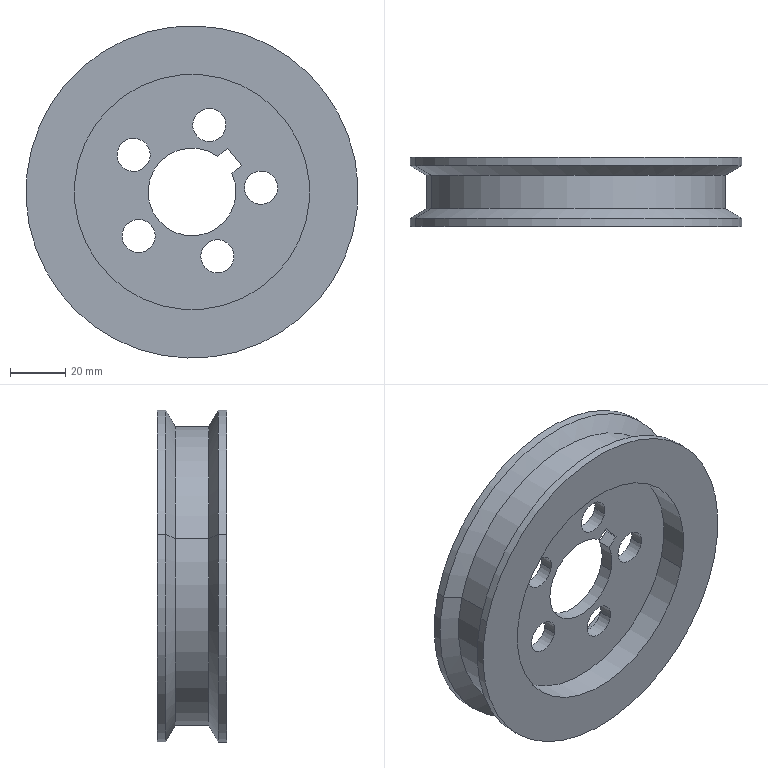Component | SolidWorks | LX-TSJ-04-1 | 1 solid | 34 faces | box 120 x 25 x 120 mm | volume 128781 mm3 | cylinder 23 | plane 7 | cone 4 | commonest cylinder face diameters 12 x10 120 x4 85 x4 31.75 x3 108 x2
STEP:
#1=CARTESIAN_POINT('',(-5.449,-19.146,-16.155));
#2=VERTEX_POINT('',#1);
#3=CARTESIAN_POINT('',(-4.238,-19.146,-16.467));
#4=VERTEX_POINT('',#3);
#5=CARTESIAN_POINT('',(-4.843,-19.146,-16.311));
#6=DIRECTION('',(0.,-1.,-0.));
#7=DIRECTION('',(0.9682,0.,-0.2502));
#8=AXIS2_PLACEMENT_3D('',#5,#6,#7);
#9=CIRCLE('',#8,0.625);
#10=EDGE_CURVE('',#2,#4,#9,.T.);
#11=ORIENTED_EDGE('',*,*,#10,.T.);
#12=CARTESIAN_POINT('',(-4.238,-18.949,-16.467));
#13=VERTEX_POINT('',#12);
#14=CARTESIAN_POINT('',(-4.238,-19.539,-16.467));
#15=DIRECTION('',(-0.,1.,0.));
#16=VECTOR('',#15,39.37);
#17=LINE('',#14,#16);
#18=EDGE_CURVE('',#4,#13,#17,.T.);
#19=ORIENTED_EDGE('',*,*,#18,.T.);
#20=CARTESIAN_POINT('',(-5.449,-18.949,-16.155));
#21=VERTEX_POINT('',#20);
#22=CARTESIAN_POINT('',(-4.843,-18.949,-16.311));
#23=DIRECTION('',(-0.,1.,0.));
#24=DIRECTION('',(-0.9682,0.,0.2502));
#25=AXIS2_PLACEMENT_3D('',#22,#23,#24);
#26=CIRCLE('',#25,0.625);
#27=EDGE_CURVE('',#13,#21,#26,.T.);
#28=ORIENTED_EDGE('',*,*,#27,.T.);
#29=CARTESIAN_POINT('',(-5.449,-19.539,-16.155));
#30=DIRECTION('',(-0.,1.,0.));
#31=VECTOR('',#30,39.37);
#32=LINE('',#29,#31);
#33=EDGE_CURVE('',#2,#21,#32,.T.);
#34=ORIENTED_EDGE('',*,*,#33,.F.);
#35=EDGE_LOOP('',(#11,#19,#28,#34));
#36=FACE_OUTER_BOUND('',#35,.T.);
#37=CARTESIAN_POINT('',(-4.843,-19.539,-16.311));
#38=DIRECTION('',(-0.,1.,0.));
#39=DIRECTION('',(-0.9682,0.,0.2502));
#40=AXIS2_PLACEMENT_3D('',#37,#38,#39);
#41=CYLINDRICAL_SURFACE('',#40,0.625);
#42=ADVANCED_FACE('',(#36),#41,.F.);
#43=CARTESIAN_POINT('',(-4.477,-19.146,-15.805));
#44=VERTEX_POINT('',#43);
#45=CARTESIAN_POINT('',(-4.843,-19.146,-16.311));
#46=DIRECTION('',(0.,-1.,-0.));
#47=DIRECTION('',(0.9682,0.,-0.2502));
#48=AXIS2_PLACEMENT_3D('',#45,#46,#47);
#49=CIRCLE('',#48,0.625);
#50=EDGE_CURVE('',#44,#2,#49,.T.);
#51=ORIENTED_EDGE('',*,*,#50,.T.);
#52=ORIENTED_EDGE('',*,*,#33,.T.);
#53=CARTESIAN_POINT('',(-4.477,-18.949,-15.805));
#54=VERTEX_POINT('',#53);
#55=CARTESIAN_POINT('',(-4.843,-18.949,-16.311));
#56=DIRECTION('',(-0.,1.,0.));
#57=DIRECTION('',(-0.9682,0.,0.2502));
#58=AXIS2_PLACEMENT_3D('',#55,#56,#57);
#59=CIRCLE('',#58,0.625);
#60=EDGE_CURVE('',#21,#54,#59,.T.);
#61=ORIENTED_EDGE('',*,*,#60,.T.);
#62=CARTESIAN_POINT('',(-4.477,-19.539,-15.805));
#63=DIRECTION('',(-0.,1.,0.));
#64=VECTOR('',#63,39.37);
#65=LINE('',#62,#64);
#66=EDGE_CURVE('',#44,#54,#65,.T.);
#67=ORIENTED_EDGE('',*,*,#66,.F.);
#68=EDGE_LOOP('',(#51,#52,#61,#67));
#69=FACE_OUTER_BOUND('',#68,.T.);
#70=CARTESIAN_POINT('',(-4.843,-19.539,-16.311));
#71=DIRECTION('',(-0.,1.,0.));
#72=DIRECTION('',(-0.9682,0.,0.2502));
#73=AXIS2_PLACEMENT_3D('',#70,#71,#72);
#74=CYLINDRICAL_SURFACE('',#73,0.625);
#75=ADVANCED_FACE('',(#69),#74,.F.);
#76=CARTESIAN_POINT('',(-7.13,-18.555,-15.72));
#77=VERTEX_POINT('',#76);
#78=CARTESIAN_POINT('',(-2.556,-18.555,-16.902));
#79=VERTEX_POINT('',#78);
#80=CARTESIAN_POINT('',(-4.843,-18.555,-16.311));
#81=DIRECTION('',(-0.,1.,0.));
#82=DIRECTION('',(0.9682,0.,-0.2502));
#83=AXIS2_PLACEMENT_3D('',#80,#81,#82);
#84=CIRCLE('',#83,2.362);
#85=EDGE_CURVE('',#77,#79,#84,.T.);
#86=ORIENTED_EDGE('',*,*,#85,.F.);
#87=CARTESIAN_POINT('',(-7.13,-18.673,-15.72));
#88=VERTEX_POINT('',#87);
#89=CARTESIAN_POINT('',(-7.13,-18.555,-15.72));
#90=DIRECTION('',(0.,-1.,-0.));
#91=VECTOR('',#90,39.37);
#92=LINE('',#89,#91);
#93=EDGE_CURVE('',#77,#88,#92,.T.);
#94=ORIENTED_EDGE('',*,*,#93,.T.);
#95=CARTESIAN_POINT('',(-2.556,-18.673,-16.902));
#96=VERTEX_POINT('',#95);
#97=CARTESIAN_POINT('',(-4.843,-18.673,-16.311));
#98=DIRECTION('',(-0.,1.,0.));
#99=DIRECTION('',(0.9682,0.,-0.2502));
#100=AXIS2_PLACEMENT_3D('',#97,#98,#99);
#101=CIRCLE('',#100,2.362);
#102=EDGE_CURVE('',#88,#96,#101,.T.);
#103=ORIENTED_EDGE('',*,*,#102,.T.);
#104=CARTESIAN_POINT('',(-2.556,-18.555,-16.902));
#105=DIRECTION('',(0.,-1.,-0.));
#106=VECTOR('',#105,39.37);
#107=LINE('',#104,#106);
#108=EDGE_CURVE('',#79,#96,#107,.T.);
#109=ORIENTED_EDGE('',*,*,#108,.F.);
#110=EDGE_LOOP('',(#86,#94,#103,#109));
#111=FACE_OUTER_BOUND('',#110,.T.);
#112=CARTESIAN_POINT('',(-4.843,-18.555,-16.311));
#113=DIRECTION('',(0.,-1.,-0.));
#114=DIRECTION('',(0.9682,0.,-0.2502));
#115=AXIS2_PLACEMENT_3D('',#112,#113,#114);
#116=CYLINDRICAL_SURFACE('',#115,2.362);
#117=ADVANCED_FACE('',(#111),#116,.T.);
#118=CARTESIAN_POINT('',(-3.223,-18.949,-16.73));
#119=VERTEX_POINT('',#118);
#120=CARTESIAN_POINT('',(-6.463,-18.949,-15.892));
#121=VERTEX_POINT('',#120);
#122=CARTESIAN_POINT('',(-4.843,-18.949,-16.311));
#123=DIRECTION('',(-0.,1.,0.));
#124=DIRECTION('',(-0.9682,-0.,0.2502));
#125=AXIS2_PLACEMENT_3D('',#122,#123,#124);
#126=CIRCLE('',#125,1.673);
#127=EDGE_CURVE('',#119,#121,#126,.T.);
#128=ORIENTED_EDGE('',*,*,#127,.F.);
#129=CARTESIAN_POINT('',(-3.223,-18.555,-16.73));
#130=VERTEX_POINT('',#129);
#131=CARTESIAN_POINT('',(-3.223,-18.949,-16.73));
#132=DIRECTION('',(-0.,1.,0.));
#133=VECTOR('',#132,39.37);
#134=LINE('',#131,#133);
#135=EDGE_CURVE('',#119,#130,#134,.T.);
#136=ORIENTED_EDGE('',*,*,#135,.T.);
#137=CARTESIAN_POINT('',(-6.463,-18.555,-15.892));
#138=VERTEX_POINT('',#137);
#139=CARTESIAN_POINT('',(-4.843,-18.555,-16.311));
#140=DIRECTION('',(0.,-1.,-0.));
#141=DIRECTION('',(-0.9682,-0.,0.2502));
#142=AXIS2_PLACEMENT_3D('',#139,#140,#141);
#143=CIRCLE('',#142,1.673);
#144=EDGE_CURVE('',#138,#130,#143,.T.);
#145=ORIENTED_EDGE('',*,*,#144,.F.);
#146=CARTESIAN_POINT('',(-6.463,-18.949,-15.892));
#147=DIRECTION('',(-0.,1.,0.));
#148=VECTOR('',#147,39.37);
#149=LINE('',#146,#148);
#150=EDGE_CURVE('',#121,#138,#149,.T.);
#151=ORIENTED_EDGE('',*,*,#150,.F.);
#152=EDGE_LOOP('',(#128,#136,#145,#151));
#153=FACE_OUTER_BOUND('',#152,.T.);
#154=CARTESIAN_POINT('',(-4.843,-18.949,-16.311));
#155=DIRECTION('',(-0.,1.,0.));
#156=DIRECTION('',(-0.9682,-0.,0.2502));
#157=AXIS2_PLACEMENT_3D('',#154,#155,#156);
#158=CYLINDRICAL_SURFACE('',#157,1.673);
#159=ADVANCED_FACE('',(#153),#158,.F.);
#160=CARTESIAN_POINT('',(-6.902,-18.81,-15.779));
#161=VERTEX_POINT('',#160);
#162=CARTESIAN_POINT('',(-2.785,-18.81,-16.843));
#163=VERTEX_POINT('',#162);
#164=CARTESIAN_POINT('',(-4.843,-18.81,-16.311));
#165=DIRECTION('',(-0.,1.,0.));
#166=DIRECTION('',(-0.9682,-0.,0.2502));
#167=AXIS2_PLACEMENT_3D('',#164,#165,#166);
#168=CIRCLE('',#167,2.126);
#169=EDGE_CURVE('',#161,#163,#168,.T.);
#170=ORIENTED_EDGE('',*,*,#169,.T.);
#171=CARTESIAN_POINT('',(-2.556,-18.673,-16.902));
#172=DIRECTION('',(0.8385,0.5,-0.2167));
#173=VECTOR('',#172,39.37);
#174=LINE('',#171,#173);
#175=EDGE_CURVE('',#163,#96,#174,.T.);
#176=ORIENTED_EDGE('',*,*,#175,.T.);
#177=ORIENTED_EDGE('',*,*,#102,.F.);
#178=CARTESIAN_POINT('',(-7.13,-18.673,-15.72));
#179=DIRECTION('',(-0.8385,0.5,0.2167));
#180=VECTOR('',#179,39.37);
#181=LINE('',#178,#180);
#182=EDGE_CURVE('',#161,#88,#181,.T.);
#183=ORIENTED_EDGE('',*,*,#182,.F.);
#184=EDGE_LOOP('',(#170,#176,#177,#183));
#185=FACE_OUTER_BOUND('',#184,.T.);
#186=CARTESIAN_POINT('',(-4.843,-18.673,-16.311));
#187=DIRECTION('',(-0.,1.,0.));
#188=DIRECTION('',(-0.9682,-0.,0.2502));
#189=AXIS2_PLACEMENT_3D('',#186,#187,#188);
#190=CONICAL_SURFACE('',#189,2.362,1.047);
#191=ADVANCED_FACE('',(#185),#190,.T.);
#192=CARTESIAN_POINT('',(-6.902,-19.285,-15.779));
#193=VERTEX_POINT('',#192);
#194=CARTESIAN_POINT('',(-2.785,-19.285,-16.843));
#195=VERTEX_POINT('',#194);
#196=CARTESIAN_POINT('',(-4.843,-19.285,-16.311));
#197=DIRECTION('',(-0.,1.,0.));
#198=DIRECTION('',(-0.9682,-0.,0.2502));
#199=AXIS2_PLACEMENT_3D('',#196,#197,#198);
#200=CIRCLE('',#199,2.126);
#201=EDGE_CURVE('',#193,#195,#200,.T.);
#202=ORIENTED_EDGE('',*,*,#201,.T.);
#203=CARTESIAN_POINT('',(-2.785,-19.047,-16.843));
#204=DIRECTION('',(-0.,1.,0.));
#205=VECTOR('',#204,39.37);
#206=LINE('',#203,#205);
#207=EDGE_CURVE('',#195,#163,#206,.T.);
#208=ORIENTED_EDGE('',*,*,#207,.T.);
#209=ORIENTED_EDGE('',*,*,#169,.F.);
#210=CARTESIAN_POINT('',(-6.902,-19.047,-15.779));
#211=DIRECTION('',(-0.,1.,0.));
#212=VECTOR('',#211,39.37);
#213=LINE('',#210,#212);
#214=EDGE_CURVE('',#193,#161,#213,.T.);
#215=ORIENTED_EDGE('',*,*,#214,.F.);
#216=EDGE_LOOP('',(#202,#208,#209,#215));
#217=FACE_OUTER_BOUND('',#216,.T.);
#218=CARTESIAN_POINT('',(-4.843,-19.047,-16.311));
#219=DIRECTION('',(-0.,1.,0.));
#220=DIRECTION('',(-0.9682,-0.,0.2502));
#221=AXIS2_PLACEMENT_3D('',#218,#219,#220);
#222=CYLINDRICAL_SURFACE('',#221,2.126);
#223=ADVANCED_FACE('',(#217),#222,.T.);
#224=CARTESIAN_POINT('',(-4.368,-19.146,-15.417));
#225=VERTEX_POINT('',#224);
#226=CARTESIAN_POINT('',(-4.826,-19.146,-15.299));
#227=VERTEX_POINT('',#226);
#228=CARTESIAN_POINT('',(-4.597,-19.146,-15.358));
#229=DIRECTION('',(-0.,1.,0.));
#230=DIRECTION('',(-0.9682,0.,0.2502));
#231=AXIS2_PLACEMENT_3D('',#228,#229,#230);
#232=CIRCLE('',#231,0.2362);
#233=EDGE_CURVE('',#225,#227,#232,.T.);
#234=ORIENTED_EDGE('',*,*,#233,.F.);
#235=CARTESIAN_POINT('',(-4.368,-18.949,-15.417));
#236=VERTEX_POINT('',#235);
#237=CARTESIAN_POINT('',(-4.368,-19.539,-15.417));
#238=DIRECTION('',(-0.,1.,0.));
#239=VECTOR('',#238,39.37);
#240=LINE('',#237,#239);
#241=EDGE_CURVE('',#225,#236,#240,.T.);
#242=ORIENTED_EDGE('',*,*,#241,.T.);
#243=CARTESIAN_POINT('',(-4.826,-18.949,-15.299));
#244=VERTEX_POINT('',#243);
#245=CARTESIAN_POINT('',(-4.597,-18.949,-15.358));
#246=DIRECTION('',(0.,-1.,-0.));
#247=DIRECTION('',(-0.9682,0.,0.2502));
#248=AXIS2_PLACEMENT_3D('',#245,#246,#247);
#249=CIRCLE('',#248,0.2362);
#250=EDGE_CURVE('',#244,#236,#249,.T.);
#251=ORIENTED_EDGE('',*,*,#250,.F.);
#252=CARTESIAN_POINT('',(-4.826,-19.539,-15.299));
#253=DIRECTION('',(-0.,1.,0.));
#254=VECTOR('',#253,39.37);
#255=LINE('',#252,#254);
#256=EDGE_CURVE('',#227,#244,#255,.T.);
#257=ORIENTED_EDGE('',*,*,#256,.F.);
#258=EDGE_LOOP('',(#234,#242,#251,#257));
#259=FACE_OUTER_BOUND('',#258,.T.);
#260=CARTESIAN_POINT('',(-4.597,-19.539,-15.358));
#261=DIRECTION('',(-0.,1.,0.));
#262=DIRECTION('',(-0.9682,0.,0.2502));
#263=AXIS2_PLACEMENT_3D('',#260,#261,#262);
#264=CYLINDRICAL_SURFACE('',#263,0.2362);
#265=ADVANCED_FACE('',(#259),#264,.F.);
#266=CARTESIAN_POINT('',(-3.632,-19.146,-16.31));
#267=VERTEX_POINT('',#266);
#268=CARTESIAN_POINT('',(-4.09,-19.146,-16.192));
#269=VERTEX_POINT('',#268);
#270=CARTESIAN_POINT('',(-3.861,-19.146,-16.251));
#271=DIRECTION('',(-0.,1.,0.));
#272=DIRECTION('',(-0.9682,0.,0.2502));
#273=AXIS2_PLACEMENT_3D('',#270,#271,#272);
#274=CIRCLE('',#273,0.2362);
#275=EDGE_CURVE('',#267,#269,#274,.T.);
#276=ORIENTED_EDGE('',*,*,#275,.F.);
#277=CARTESIAN_POINT('',(-3.632,-18.949,-16.31));
#278=VERTEX_POINT('',#277);
#279=CARTESIAN_POINT('',(-3.632,-19.539,-16.31));
#280=DIRECTION('',(-0.,1.,0.));
#281=VECTOR('',#280,39.37);
#282=LINE('',#279,#281);
#283=EDGE_CURVE('',#267,#278,#282,.T.);
#284=ORIENTED_EDGE('',*,*,#283,.T.);
#285=CARTESIAN_POINT('',(-4.09,-18.949,-16.192));
#286=VERTEX_POINT('',#285);
#287=CARTESIAN_POINT('',(-3.861,-18.949,-16.251));
#288=DIRECTION('',(0.,-1.,-0.));
#289=DIRECTION('',(-0.9682,0.,0.2502));
#290=AXIS2_PLACEMENT_3D('',#287,#288,#289);
#291=CIRCLE('',#290,0.2362);
#292=EDGE_CURVE('',#286,#278,#291,.T.);
#293=ORIENTED_EDGE('',*,*,#292,.F.);
#294=CARTESIAN_POINT('',(-4.09,-19.539,-16.192));
#295=DIRECTION('',(-0.,1.,0.));
#296=VECTOR('',#295,39.37);
#297=LINE('',#294,#296);
#298=EDGE_CURVE('',#269,#286,#297,.T.);
#299=ORIENTED_EDGE('',*,*,#298,.F.);
#300=EDGE_LOOP('',(#276,#284,#293,#299));
#301=FACE_OUTER_BOUND('',#300,.T.);
#302=CARTESIAN_POINT('',(-3.861,-19.539,-16.251));
#303=DIRECTION('',(-0.,1.,0.));
#304=DIRECTION('',(-0.9682,0.,0.2502));
#305=AXIS2_PLACEMENT_3D('',#302,#303,#304);
#306=CYLINDRICAL_SURFACE('',#305,0.2362);
#307=ADVANCED_FACE('',(#301),#306,.F.);
#308=CARTESIAN_POINT('',(-4.254,-19.146,-17.286));
#309=VERTEX_POINT('',#308);
#310=CARTESIAN_POINT('',(-4.711,-19.146,-17.168));
#311=VERTEX_POINT('',#310);
#312=CARTESIAN_POINT('',(-4.482,-19.146,-17.227));
#313=DIRECTION('',(-0.,1.,0.));
#314=DIRECTION('',(-0.9682,0.,0.2502));
#315=AXIS2_PLACEMENT_3D('',#312,#313,#314);
#316=CIRCLE('',#315,0.2362);
#317=EDGE_CURVE('',#309,#311,#316,.T.);
#318=ORIENTED_EDGE('',*,*,#317,.F.);
#319=CARTESIAN_POINT('',(-4.254,-18.949,-17.286));
#320=VERTEX_POINT('',#319);
#321=CARTESIAN_POINT('',(-4.254,-19.539,-17.286));
#322=DIRECTION('',(-0.,1.,0.));
#323=VECTOR('',#322,39.37);
#324=LINE('',#321,#323);
#325=EDGE_CURVE('',#309,#320,#324,.T.);
#326=ORIENTED_EDGE('',*,*,#325,.T.);
#327=CARTESIAN_POINT('',(-4.711,-18.949,-17.168));
#328=VERTEX_POINT('',#327);
#329=CARTESIAN_POINT('',(-4.482,-18.949,-17.227));
#330=DIRECTION('',(0.,-1.,-0.));
#331=DIRECTION('',(-0.9682,0.,0.2502));
#332=AXIS2_PLACEMENT_3D('',#329,#330,#331);
#333=CIRCLE('',#332,0.2362);
#334=EDGE_CURVE('',#328,#320,#333,.T.);
#335=ORIENTED_EDGE('',*,*,#334,.F.);
#336=CARTESIAN_POINT('',(-4.711,-19.539,-17.168));
#337=DIRECTION('',(-0.,1.,0.));
#338=VECTOR('',#337,39.37);
#339=LINE('',#336,#338);
#340=EDGE_CURVE('',#311,#328,#339,.T.);
#341=ORIENTED_EDGE('',*,*,#340,.F.);
#342=EDGE_LOOP('',(#318,#326,#335,#341));
#343=FACE_OUTER_BOUND('',#342,.T.);
#344=CARTESIAN_POINT('',(-4.482,-19.539,-17.227));
#345=DIRECTION('',(-0.,1.,0.));
#346=DIRECTION('',(-0.9682,0.,0.2502));
#347=AXIS2_PLACEMENT_3D('',#344,#345,#346);
#348=CYLINDRICAL_SURFACE('',#347,0.2362);
#349=ADVANCED_FACE('',(#343),#348,.F.);
#350=CARTESIAN_POINT('',(-5.374,-19.146,-16.996));
#351=VERTEX_POINT('',#350);
#352=CARTESIAN_POINT('',(-5.831,-19.146,-16.878));
#353=VERTEX_POINT('',#352);
#354=CARTESIAN_POINT('',(-5.603,-19.146,-16.937));
#355=DIRECTION('',(-0.,1.,0.));
#356=DIRECTION('',(-0.9682,0.,0.2502));
#357=AXIS2_PLACEMENT_3D('',#354,#355,#356);
#358=CIRCLE('',#357,0.2362);
#359=EDGE_CURVE('',#351,#353,#358,.T.);
#360=ORIENTED_EDGE('',*,*,#359,.F.);
#361=CARTESIAN_POINT('',(-5.374,-18.949,-16.996));
#362=VERTEX_POINT('',#361);
#363=CARTESIAN_POINT('',(-5.374,-19.539,-16.996));
#364=DIRECTION('',(-0.,1.,0.));
#365=VECTOR('',#364,39.37);
#366=LINE('',#363,#365);
#367=EDGE_CURVE('',#351,#362,#366,.T.);
#368=ORIENTED_EDGE('',*,*,#367,.T.);
#369=CARTESIAN_POINT('',(-5.831,-18.949,-16.878));
#370=VERTEX_POINT('',#369);
#371=CARTESIAN_POINT('',(-5.603,-18.949,-16.937));
#372=DIRECTION('',(0.,-1.,-0.));
#373=DIRECTION('',(-0.9682,0.,0.2502));
#374=AXIS2_PLACEMENT_3D('',#371,#372,#373);
#375=CIRCLE('',#374,0.2362);
#376=EDGE_CURVE('',#370,#362,#375,.T.);
#377=ORIENTED_EDGE('',*,*,#376,.F.);
#378=CARTESIAN_POINT('',(-5.831,-19.539,-16.878));
#379=DIRECTION('',(-0.,1.,0.));
#380=VECTOR('',#379,39.37);
#381=LINE('',#378,#380);
#382=EDGE_CURVE('',#353,#370,#381,.T.);
#383=ORIENTED_EDGE('',*,*,#382,.F.);
#384=EDGE_LOOP('',(#360,#368,#377,#383));
#385=FACE_OUTER_BOUND('',#384,.T.);
#386=CARTESIAN_POINT('',(-5.603,-19.539,-16.937));
#387=DIRECTION('',(-0.,1.,0.));
#388=DIRECTION('',(-0.9682,0.,0.2502));
#389=AXIS2_PLACEMENT_3D('',#386,#387,#388);
#390=CYLINDRICAL_SURFACE('',#389,0.2362);
#391=ADVANCED_FACE('',(#385),#390,.F.);
#392=CARTESIAN_POINT('',(-5.445,-19.146,-15.841));
#393=VERTEX_POINT('',#392);
#394=CARTESIAN_POINT('',(-5.902,-19.146,-15.723));
#395=VERTEX_POINT('',#394);
#396=CARTESIAN_POINT('',(-5.674,-19.146,-15.782));
#397=DIRECTION('',(-0.,1.,0.));
#398=DIRECTION('',(-0.9682,0.,0.2502));
#399=AXIS2_PLACEMENT_3D('',#396,#397,#398);
#400=CIRCLE('',#399,0.2362);
#401=EDGE_CURVE('',#393,#395,#400,.T.);
#402=ORIENTED_EDGE('',*,*,#401,.F.);
#403=CARTESIAN_POINT('',(-5.445,-18.949,-15.841));
#404=VERTEX_POINT('',#403);
#405=CARTESIAN_POINT('',(-5.445,-19.539,-15.841));
#406=DIRECTION('',(-0.,1.,0.));
#407=VECTOR('',#406,39.37);
#408=LINE('',#405,#407);
#409=EDGE_CURVE('',#393,#404,#408,.T.);
#410=ORIENTED_EDGE('',*,*,#409,.T.);
#411=CARTESIAN_POINT('',(-5.902,-18.949,-15.723));
#412=VERTEX_POINT('',#411);
#413=CARTESIAN_POINT('',(-5.674,-18.949,-15.782));
#414=DIRECTION('',(0.,-1.,-0.));
#415=DIRECTION('',(-0.9682,0.,0.2502));
#416=AXIS2_PLACEMENT_3D('',#413,#414,#415);
#417=CIRCLE('',#416,0.2362);
#418=EDGE_CURVE('',#412,#404,#417,.T.);
#419=ORIENTED_EDGE('',*,*,#418,.F.);
#420=CARTESIAN_POINT('',(-5.902,-19.539,-15.723));
#421=DIRECTION('',(-0.,1.,0.));
#422=VECTOR('',#421,39.37);
#423=LINE('',#420,#422);
#424=EDGE_CURVE('',#395,#412,#423,.T.);
#425=ORIENTED_EDGE('',*,*,#424,.F.);
#426=EDGE_LOOP('',(#402,#410,#419,#425));
#427=FACE_OUTER_BOUND('',#426,.T.);
#428=CARTESIAN_POINT('',(-5.674,-19.539,-15.782));
#429=DIRECTION('',(-0.,1.,0.));
#430=DIRECTION('',(-0.9682,0.,0.2502));
#431=AXIS2_PLACEMENT_3D('',#428,#429,#430);
#432=CYLINDRICAL_SURFACE('',#431,0.2362);
#433=ADVANCED_FACE('',(#427),#432,.F.);
#434=ORIENTED_EDGE('',*,*,#201,.F.);
#435=CARTESIAN_POINT('',(-7.13,-19.421,-15.72));
#436=VERTEX_POINT('',#435);
#437=CARTESIAN_POINT('',(-7.13,-19.421,-15.72));
#438=DIRECTION('',(-0.8385,-0.5,0.2167));
#439=VECTOR('',#438,39.37);
#440=LINE('',#437,#439);
#441=EDGE_CURVE('',#193,#436,#440,.T.);
#442=ORIENTED_EDGE('',*,*,#441,.T.);
#443=CARTESIAN_POINT('',(-2.556,-19.421,-16.902));
#444=VERTEX_POINT('',#443);
#445=CARTESIAN_POINT('',(-4.843,-19.421,-16.311));
#446=DIRECTION('',(-0.,1.,0.));
#447=DIRECTION('',(0.9682,0.,-0.2502));
#448=AXIS2_PLACEMENT_3D('',#445,#446,#447);
#449=CIRCLE('',#448,2.362);
#450=EDGE_CURVE('',#436,#444,#449,.T.);
#451=ORIENTED_EDGE('',*,*,#450,.T.);
#452=CARTESIAN_POINT('',(-2.556,-19.421,-16.902));
#453=DIRECTION('',(0.8385,-0.5,-0.2167));
#454=VECTOR('',#453,39.37);
#455=LINE('',#452,#454);
#456=EDGE_CURVE('',#195,#444,#455,.T.);
#457=ORIENTED_EDGE('',*,*,#456,.F.);
#458=EDGE_LOOP('',(#434,#442,#451,#457));
#459=FACE_OUTER_BOUND('',#458,.T.);
#460=CARTESIAN_POINT('',(-4.843,-19.421,-16.311));
#461=DIRECTION('',(0.,-1.,-0.));
#462=DIRECTION('',(0.9682,0.,-0.2502));
#463=AXIS2_PLACEMENT_3D('',#460,#461,#462);
#464=CONICAL_SURFACE('',#463,2.362,1.047);
#465=ADVANCED_FACE('',(#459),#464,.T.);
#466=ORIENTED_EDGE('',*,*,#450,.F.);
#467=CARTESIAN_POINT('',(-7.13,-19.539,-15.72));
#468=VERTEX_POINT('',#467);
#469=CARTESIAN_POINT('',(-7.13,-18.555,-15.72));
#470=DIRECTION('',(0.,-1.,-0.));
#471=VECTOR('',#470,39.37);
#472=LINE('',#469,#471);
#473=EDGE_CURVE('',#436,#468,#472,.T.);
#474=ORIENTED_EDGE('',*,*,#473,.T.);
#475=CARTESIAN_POINT('',(-2.556,-19.539,-16.902));
#476=VERTEX_POINT('',#475);
#477=CARTESIAN_POINT('',(-4.843,-19.539,-16.311));
#478=DIRECTION('',(-0.,1.,0.));
#479=DIRECTION('',(0.9682,0.,-0.2502));
#480=AXIS2_PLACEMENT_3D('',#477,#478,#479);
#481=CIRCLE('',#480,2.362);
#482=EDGE_CURVE('',#468,#476,#481,.T.);
#483=ORIENTED_EDGE('',*,*,#482,.T.);
#484=CARTESIAN_POINT('',(-2.556,-18.555,-16.902));
#485=DIRECTION('',(0.,-1.,-0.));
#486=VECTOR('',#485,39.37);
#487=LINE('',#484,#486);
#488=EDGE_CURVE('',#444,#476,#487,.T.);
#489=ORIENTED_EDGE('',*,*,#488,.F.);
#490=EDGE_LOOP('',(#466,#474,#483,#489));
#491=FACE_OUTER_BOUND('',#490,.T.);
#492=CARTESIAN_POINT('',(-4.843,-18.555,-16.311));
#493=DIRECTION('',(0.,-1.,-0.));
#494=DIRECTION('',(0.9682,0.,-0.2502));
#495=AXIS2_PLACEMENT_3D('',#492,#493,#494);
#496=CYLINDRICAL_SURFACE('',#495,2.362);
#497=ADVANCED_FACE('',(#491),#496,.T.);
#498=CARTESIAN_POINT('',(-6.463,-19.146,-15.892));
#499=VERTEX_POINT('',#498);
#500=CARTESIAN_POINT('',(-3.223,-19.146,-16.73));
#501=VERTEX_POINT('',#500);
#502=CARTESIAN_POINT('',(-4.843,-19.146,-16.311));
#503=DIRECTION('',(0.,-1.,-0.));
#504=DIRECTION('',(0.9682,0.,-0.2502));
#505=AXIS2_PLACEMENT_3D('',#502,#503,#504);
#506=CIRCLE('',#505,1.673);
#507=EDGE_CURVE('',#499,#501,#506,.T.);
#508=ORIENTED_EDGE('',*,*,#507,.F.);
#509=CARTESIAN_POINT('',(-6.463,-19.539,-15.892));
#510=VERTEX_POINT('',#509);
#511=CARTESIAN_POINT('',(-6.463,-19.146,-15.892));
#512=DIRECTION('',(0.,-1.,-0.));
#513=VECTOR('',#512,39.37);
#514=LINE('',#511,#513);
#515=EDGE_CURVE('',#499,#510,#514,.T.);
#516=ORIENTED_EDGE('',*,*,#515,.T.);
#517=CARTESIAN_POINT('',(-3.223,-19.539,-16.73));
#518=VERTEX_POINT('',#517);
#519=CARTESIAN_POINT('',(-4.843,-19.539,-16.311));
#520=DIRECTION('',(-0.,1.,0.));
#521=DIRECTION('',(0.9682,0.,-0.2502));
#522=AXIS2_PLACEMENT_3D('',#519,#520,#521);
#523=CIRCLE('',#522,1.673);
#524=EDGE_CURVE('',#518,#510,#523,.T.);
#525=ORIENTED_EDGE('',*,*,#524,.F.);
#526=CARTESIAN_POINT('',(-3.223,-19.146,-16.73));
#527=DIRECTION('',(0.,-1.,-0.));
#528=VECTOR('',#527,39.37);
#529=LINE('',#526,#528);
#530=EDGE_CURVE('',#501,#518,#529,.T.);
#531=ORIENTED_EDGE('',*,*,#530,.F.);
#532=EDGE_LOOP('',(#508,#516,#525,#531));
#533=FACE_OUTER_BOUND('',#532,.T.);
#534=CARTESIAN_POINT('',(-4.843,-19.146,-16.311));
#535=DIRECTION('',(0.,-1.,-0.));
#536=DIRECTION('',(0.9682,0.,-0.2502));
#537=AXIS2_PLACEMENT_3D('',#534,#535,#536);
#538=CYLINDRICAL_SURFACE('',#537,1.673);
#539=ADVANCED_FACE('',(#533),#538,.F.);
#540=CARTESIAN_POINT('',(-4.843,-18.555,-16.311));
#541=DIRECTION('',(-0.,1.,0.));
#542=DIRECTION('',(0.9682,0.,-0.2502));
#543=AXIS2_PLACEMENT_3D('',#540,#541,#542);
#544=CIRCLE('',#543,2.362);
#545=EDGE_CURVE('',#79,#77,#544,.T.);
#546=ORIENTED_EDGE('',*,*,#545,.T.);
#547=ORIENTED_EDGE('',*,*,#85,.T.);
#548=EDGE_LOOP('',(#546,#547));
#549=FACE_OUTER_BOUND('',#548,.T.);
#550=ORIENTED_EDGE('',*,*,#144,.T.);
#551=CARTESIAN_POINT('',(-4.843,-18.555,-16.311));
#552=DIRECTION('',(0.,-1.,-0.));
#553=DIRECTION('',(-0.9682,-0.,0.2502));
#554=AXIS2_PLACEMENT_3D('',#551,#552,#553);
#555=CIRCLE('',#554,1.673);
#556=EDGE_CURVE('',#130,#138,#555,.T.);
#557=ORIENTED_EDGE('',*,*,#556,.T.);
#558=EDGE_LOOP('',(#550,#557));
#559=FACE_BOUND('',#558,.T.);
#560=CARTESIAN_POINT('',(-4.843,-18.555,-16.311));
#561=DIRECTION('',(-0.,1.,0.));
#562=DIRECTION('',(-0.9682,-0.,0.2502));
#563=AXIS2_PLACEMENT_3D('',#560,#561,#562);
#564=PLANE('',#563);
#565=ADVANCED_FACE('',(#549,#559),#564,.T.);
#566=ORIENTED_EDGE('',*,*,#93,.F.);
#567=ORIENTED_EDGE('',*,*,#545,.F.);
#568=ORIENTED_EDGE('',*,*,#108,.T.);
#569=CARTESIAN_POINT('',(-4.843,-18.673,-16.311));
#570=DIRECTION('',(-0.,1.,0.));
#571=DIRECTION('',(0.9682,0.,-0.2502));
#572=AXIS2_PLACEMENT_3D('',#569,#570,#571);
#573=CIRCLE('',#572,2.362);
#574=EDGE_CURVE('',#96,#88,#573,.T.);
#575=ORIENTED_EDGE('',*,*,#574,.T.);
#576=EDGE_LOOP('',(#566,#567,#568,#575));
#577=FACE_OUTER_BOUND('',#576,.T.);
#578=CARTESIAN_POINT('',(-4.843,-18.555,-16.311));
#579=DIRECTION('',(0.,-1.,-0.));
#580=DIRECTION('',(0.9682,0.,-0.2502));
#581=AXIS2_PLACEMENT_3D('',#578,#579,#580);
#582=CYLINDRICAL_SURFACE('',#581,2.362);
#583=ADVANCED_FACE('',(#577),#582,.T.);
#584=ORIENTED_EDGE('',*,*,#135,.F.);
#585=CARTESIAN_POINT('',(-4.843,-18.949,-16.311));
#586=DIRECTION('',(-0.,1.,0.));
#587=DIRECTION('',(-0.9682,-0.,0.2502));
#588=AXIS2_PLACEMENT_3D('',#585,#586,#587);
#589=CIRCLE('',#588,1.673);
#590=EDGE_CURVE('',#121,#119,#589,.T.);
#591=ORIENTED_EDGE('',*,*,#590,.F.);
#592=ORIENTED_EDGE('',*,*,#150,.T.);
#593=ORIENTED_EDGE('',*,*,#556,.F.);
#594=EDGE_LOOP('',(#584,#591,#592,#593));
#595=FACE_OUTER_BOUND('',#594,.T.);
#596=CARTESIAN_POINT('',(-4.843,-18.949,-16.311));
#597=DIRECTION('',(-0.,1.,0.));
#598=DIRECTION('',(-0.9682,-0.,0.2502));
#599=AXIS2_PLACEMENT_3D('',#596,#597,#598);
#600=CYLINDRICAL_SURFACE('',#599,1.673);
#601=ADVANCED_FACE('',(#595),#600,.F.);
#602=ORIENTED_EDGE('',*,*,#175,.F.);
#603=CARTESIAN_POINT('',(-4.843,-18.81,-16.311));
#604=DIRECTION('',(-0.,1.,0.));
#605=DIRECTION('',(-0.9682,-0.,0.2502));
#606=AXIS2_PLACEMENT_3D('',#603,#604,#605);
#607=CIRCLE('',#606,2.126);
#608=EDGE_CURVE('',#163,#161,#607,.T.);
#609=ORIENTED_EDGE('',*,*,#608,.T.);
#610=ORIENTED_EDGE('',*,*,#182,.T.);
#611=ORIENTED_EDGE('',*,*,#574,.F.);
#612=EDGE_LOOP('',(#602,#609,#610,#611));
#613=FACE_OUTER_BOUND('',#612,.T.);
#614=CARTESIAN_POINT('',(-4.843,-18.673,-16.311));
#615=DIRECTION('',(-0.,1.,0.));
#616=DIRECTION('',(-0.9682,-0.,0.2502));
#617=AXIS2_PLACEMENT_3D('',#614,#615,#616);
#618=CONICAL_SURFACE('',#617,2.362,1.047);
#619=ADVANCED_FACE('',(#613),#618,.T.);
#620=CARTESIAN_POINT('',(-4.277,-18.949,-16.048));
#621=VERTEX_POINT('',#620);
#622=CARTESIAN_POINT('',(-4.843,-18.949,-16.311));
#623=DIRECTION('',(-0.,1.,0.));
#624=DIRECTION('',(-0.9682,0.,0.2502));
#625=AXIS2_PLACEMENT_3D('',#622,#623,#624);
#626=CIRCLE('',#625,0.625);
#627=EDGE_CURVE('',#621,#13,#626,.T.);
#628=ORIENTED_EDGE('',*,*,#627,.F.);
#629=CARTESIAN_POINT('',(-4.136,-18.949,-15.931));
#630=VERTEX_POINT('',#629);
#631=CARTESIAN_POINT('',(-4.288,-18.949,-16.057));
#632=DIRECTION('',(0.7715,-0.,0.6362));
#633=VECTOR('',#632,39.37);
#634=LINE('',#631,#633);
#635=EDGE_CURVE('',#621,#630,#634,.T.);
#636=ORIENTED_EDGE('',*,*,#635,.T.);
#637=CARTESIAN_POINT('',(-4.336,-18.949,-15.688));
#638=VERTEX_POINT('',#637);
#639=CARTESIAN_POINT('',(-4.136,-18.949,-15.931));
#640=DIRECTION('',(-0.6362,-0.,0.7715));
#641=VECTOR('',#640,39.37);
#642=LINE('',#639,#641);
#643=EDGE_CURVE('',#630,#638,#642,.T.);
#644=ORIENTED_EDGE('',*,*,#643,.T.);
#645=CARTESIAN_POINT('',(-4.336,-18.949,-15.688));
#646=DIRECTION('',(-0.7715,0.,-0.6362));
#647=VECTOR('',#646,39.37);
#648=LINE('',#645,#647);
#649=EDGE_CURVE('',#638,#54,#648,.T.);
#650=ORIENTED_EDGE('',*,*,#649,.T.);
#651=ORIENTED_EDGE('',*,*,#60,.F.);
#652=ORIENTED_EDGE('',*,*,#27,.F.);
#653=EDGE_LOOP('',(#628,#636,#644,#650,#651,#652));
#654=FACE_BOUND('',#653,.T.);
#655=ORIENTED_EDGE('',*,*,#590,.T.);
#656=ORIENTED_EDGE('',*,*,#127,.T.);
#657=EDGE_LOOP('',(#655,#656));
#658=FACE_OUTER_BOUND('',#657,.T.);
#659=ORIENTED_EDGE('',*,*,#250,.T.);
#660=CARTESIAN_POINT('',(-4.597,-18.949,-15.358));
#661=DIRECTION('',(0.,-1.,-0.));
#662=DIRECTION('',(-0.9682,0.,0.2502));
#663=AXIS2_PLACEMENT_3D('',#660,#661,#662);
#664=CIRCLE('',#663,0.2362);
#665=EDGE_CURVE('',#236,#244,#664,.T.);
#666=ORIENTED_EDGE('',*,*,#665,.T.);
#667=EDGE_LOOP('',(#659,#666));
#668=FACE_BOUND('',#667,.T.);
#669=ORIENTED_EDGE('',*,*,#292,.T.);
#670=CARTESIAN_POINT('',(-3.861,-18.949,-16.251));
#671=DIRECTION('',(0.,-1.,-0.));
#672=DIRECTION('',(-0.9682,0.,0.2502));
#673=AXIS2_PLACEMENT_3D('',#670,#671,#672);
#674=CIRCLE('',#673,0.2362);
#675=EDGE_CURVE('',#278,#286,#674,.T.);
#676=ORIENTED_EDGE('',*,*,#675,.T.);
#677=EDGE_LOOP('',(#669,#676));
#678=FACE_BOUND('',#677,.T.);
#679=ORIENTED_EDGE('',*,*,#334,.T.);
#680=CARTESIAN_POINT('',(-4.482,-18.949,-17.227));
#681=DIRECTION('',(0.,-1.,-0.));
#682=DIRECTION('',(-0.9682,0.,0.2502));
#683=AXIS2_PLACEMENT_3D('',#680,#681,#682);
#684=CIRCLE('',#683,0.2362);
#685=EDGE_CURVE('',#320,#328,#684,.T.);
#686=ORIENTED_EDGE('',*,*,#685,.T.);
#687=EDGE_LOOP('',(#679,#686));
#688=FACE_BOUND('',#687,.T.);
#689=ORIENTED_EDGE('',*,*,#376,.T.);
#690=CARTESIAN_POINT('',(-5.603,-18.949,-16.937));
#691=DIRECTION('',(0.,-1.,-0.));
#692=DIRECTION('',(-0.9682,0.,0.2502));
#693=AXIS2_PLACEMENT_3D('',#690,#691,#692);
#694=CIRCLE('',#693,0.2362);
#695=EDGE_CURVE('',#362,#370,#694,.T.);
#696=ORIENTED_EDGE('',*,*,#695,.T.);
#697=EDGE_LOOP('',(#689,#696));
#698=FACE_BOUND('',#697,.T.);
#699=ORIENTED_EDGE('',*,*,#418,.T.);
#700=CARTESIAN_POINT('',(-5.674,-18.949,-15.782));
#701=DIRECTION('',(0.,-1.,-0.));
#702=DIRECTION('',(-0.9682,0.,0.2502));
#703=AXIS2_PLACEMENT_3D('',#700,#701,#702);
#704=CIRCLE('',#703,0.2362);
#705=EDGE_CURVE('',#404,#412,#704,.T.);
#706=ORIENTED_EDGE('',*,*,#705,.T.);
#707=EDGE_LOOP('',(#699,#706));
#708=FACE_BOUND('',#707,.T.);
#709=CARTESIAN_POINT('',(-4.843,-18.949,-16.311));
#710=DIRECTION('',(-0.,1.,0.));
#711=DIRECTION('',(-0.9682,-0.,0.2502));
#712=AXIS2_PLACEMENT_3D('',#709,#710,#711);
#713=PLANE('',#712);
#714=ADVANCED_FACE('',(#654,#658,#668,#678,#688,#698,#708),#713,.T.);
#715=ORIENTED_EDGE('',*,*,#207,.F.);
#716=CARTESIAN_POINT('',(-4.843,-19.285,-16.311));
#717=DIRECTION('',(-0.,1.,0.));
#718=DIRECTION('',(-0.9682,-0.,0.2502));
#719=AXIS2_PLACEMENT_3D('',#716,#717,#718);
#720=CIRCLE('',#719,2.126);
#721=EDGE_CURVE('',#195,#193,#720,.T.);
#722=ORIENTED_EDGE('',*,*,#721,.T.);
#723=ORIENTED_EDGE('',*,*,#214,.T.);
#724=ORIENTED_EDGE('',*,*,#608,.F.);
#725=EDGE_LOOP('',(#715,#722,#723,#724));
#726=FACE_OUTER_BOUND('',#725,.T.);
#727=CARTESIAN_POINT('',(-4.843,-19.047,-16.311));
#728=DIRECTION('',(-0.,1.,0.));
#729=DIRECTION('',(-0.9682,-0.,0.2502));
#730=AXIS2_PLACEMENT_3D('',#727,#728,#729);
#731=CYLINDRICAL_SURFACE('',#730,2.126);
#732=ADVANCED_FACE('',(#726),#731,.T.);
#733=ORIENTED_EDGE('',*,*,#241,.F.);
#734=CARTESIAN_POINT('',(-4.597,-19.146,-15.358));
#735=DIRECTION('',(-0.,1.,0.));
#736=DIRECTION('',(-0.9682,0.,0.2502));
#737=AXIS2_PLACEMENT_3D('',#734,#735,#736);
#738=CIRCLE('',#737,0.2362);
#739=EDGE_CURVE('',#227,#225,#738,.T.);
#740=ORIENTED_EDGE('',*,*,#739,.F.);
#741=ORIENTED_EDGE('',*,*,#256,.T.);
#742=ORIENTED_EDGE('',*,*,#665,.F.);
#743=EDGE_LOOP('',(#733,#740,#741,#742));
#744=FACE_OUTER_BOUND('',#743,.T.);
#745=CARTESIAN_POINT('',(-4.597,-19.539,-15.358));
#746=DIRECTION('',(-0.,1.,0.));
#747=DIRECTION('',(-0.9682,0.,0.2502));
#748=AXIS2_PLACEMENT_3D('',#745,#746,#747);
#749=CYLINDRICAL_SURFACE('',#748,0.2362);
#750=ADVANCED_FACE('',(#744),#749,.F.);
#751=ORIENTED_EDGE('',*,*,#283,.F.);
#752=CARTESIAN_POINT('',(-3.861,-19.146,-16.251));
#753=DIRECTION('',(-0.,1.,0.));
#754=DIRECTION('',(-0.9682,0.,0.2502));
#755=AXIS2_PLACEMENT_3D('',#752,#753,#754);
#756=CIRCLE('',#755,0.2362);
#757=EDGE_CURVE('',#269,#267,#756,.T.);
#758=ORIENTED_EDGE('',*,*,#757,.F.);
#759=ORIENTED_EDGE('',*,*,#298,.T.);
#760=ORIENTED_EDGE('',*,*,#675,.F.);
#761=EDGE_LOOP('',(#751,#758,#759,#760));
#762=FACE_OUTER_BOUND('',#761,.T.);
#763=CARTESIAN_POINT('',(-3.861,-19.539,-16.251));
#764=DIRECTION('',(-0.,1.,0.));
#765=DIRECTION('',(-0.9682,0.,0.2502));
#766=AXIS2_PLACEMENT_3D('',#763,#764,#765);
#767=CYLINDRICAL_SURFACE('',#766,0.2362);
#768=ADVANCED_FACE('',(#762),#767,.F.);
#769=ORIENTED_EDGE('',*,*,#325,.F.);
#770=CARTESIAN_POINT('',(-4.482,-19.146,-17.227));
#771=DIRECTION('',(-0.,1.,0.));
#772=DIRECTION('',(-0.9682,0.,0.2502));
#773=AXIS2_PLACEMENT_3D('',#770,#771,#772);
#774=CIRCLE('',#773,0.2362);
#775=EDGE_CURVE('',#311,#309,#774,.T.);
#776=ORIENTED_EDGE('',*,*,#775,.F.);
#777=ORIENTED_EDGE('',*,*,#340,.T.);
#778=ORIENTED_EDGE('',*,*,#685,.F.);
#779=EDGE_LOOP('',(#769,#776,#777,#778));
#780=FACE_OUTER_BOUND('',#779,.T.);
#781=CARTESIAN_POINT('',(-4.482,-19.539,-17.227));
#782=DIRECTION('',(-0.,1.,0.));
#783=DIRECTION('',(-0.9682,0.,0.2502));
#784=AXIS2_PLACEMENT_3D('',#781,#782,#783);
#785=CYLINDRICAL_SURFACE('',#784,0.2362);
#786=ADVANCED_FACE('',(#780),#785,.F.);
#787=ORIENTED_EDGE('',*,*,#367,.F.);
#788=CARTESIAN_POINT('',(-5.603,-19.146,-16.937));
#789=DIRECTION('',(-0.,1.,0.));
#790=DIRECTION('',(-0.9682,0.,0.2502));
#791=AXIS2_PLACEMENT_3D('',#788,#789,#790);
#792=CIRCLE('',#791,0.2362);
#793=EDGE_CURVE('',#353,#351,#792,.T.);
#794=ORIENTED_EDGE('',*,*,#793,.F.);
#795=ORIENTED_EDGE('',*,*,#382,.T.);
#796=ORIENTED_EDGE('',*,*,#695,.F.);
#797=EDGE_LOOP('',(#787,#794,#795,#796));
#798=FACE_OUTER_BOUND('',#797,.T.);
#799=CARTESIAN_POINT('',(-5.603,-19.539,-16.937));
#800=DIRECTION('',(-0.,1.,0.));
#801=DIRECTION('',(-0.9682,0.,0.2502));
#802=AXIS2_PLACEMENT_3D('',#799,#800,#801);
#803=CYLINDRICAL_SURFACE('',#802,0.2362);
#804=ADVANCED_FACE('',(#798),#803,.F.);
#805=ORIENTED_EDGE('',*,*,#409,.F.);
#806=CARTESIAN_POINT('',(-5.674,-19.146,-15.782));
#807=DIRECTION('',(-0.,1.,0.));
#808=DIRECTION('',(-0.9682,0.,0.2502));
#809=AXIS2_PLACEMENT_3D('',#806,#807,#808);
#810=CIRCLE('',#809,0.2362);
#811=EDGE_CURVE('',#395,#393,#810,.T.);
#812=ORIENTED_EDGE('',*,*,#811,.F.);
#813=ORIENTED_EDGE('',*,*,#424,.T.);
#814=ORIENTED_EDGE('',*,*,#705,.F.);
#815=EDGE_LOOP('',(#805,#812,#813,#814));
#816=FACE_OUTER_BOUND('',#815,.T.);
#817=CARTESIAN_POINT('',(-5.674,-19.539,-15.782));
#818=DIRECTION('',(-0.,1.,0.));
#819=DIRECTION('',(-0.9682,0.,0.2502));
#820=AXIS2_PLACEMENT_3D('',#817,#818,#819);
#821=CYLINDRICAL_SURFACE('',#820,0.2362);
#822=ADVANCED_FACE('',(#816),#821,.F.);
#823=CARTESIAN_POINT('',(-4.136,-19.146,-15.931));
#824=VERTEX_POINT('',#823);
#825=CARTESIAN_POINT('',(-4.136,-18.555,-15.931));
#826=DIRECTION('',(-0.,1.,0.));
#827=VECTOR('',#826,39.37);
#828=LINE('',#825,#827);
#829=EDGE_CURVE('',#824,#630,#828,.T.);
#830=ORIENTED_EDGE('',*,*,#829,.F.);
#831=CARTESIAN_POINT('',(-4.336,-19.146,-15.688));
#832=VERTEX_POINT('',#831);
#833=CARTESIAN_POINT('',(-4.336,-19.146,-15.688));
#834=DIRECTION('',(0.6362,0.,-0.7715));
#835=VECTOR('',#834,39.37);
#836=LINE('',#833,#835);
#837=EDGE_CURVE('',#832,#824,#836,.T.);
#838=ORIENTED_EDGE('',*,*,#837,.F.);
#839=CARTESIAN_POINT('',(-4.336,-18.555,-15.688));
#840=DIRECTION('',(0.,-1.,-0.));
#841=VECTOR('',#840,39.37);
#842=LINE('',#839,#841);
#843=EDGE_CURVE('',#638,#832,#842,.T.);
#844=ORIENTED_EDGE('',*,*,#843,.F.);
#845=ORIENTED_EDGE('',*,*,#643,.F.);
#846=EDGE_LOOP('',(#830,#838,#844,#845));
#847=FACE_OUTER_BOUND('',#846,.T.);
#848=CARTESIAN_POINT('',(-4.336,-18.555,-15.688));
#849=DIRECTION('',(0.7715,-0.,0.6362));
#850=DIRECTION('',(0.6362,0.,-0.7715));
#851=AXIS2_PLACEMENT_3D('',#848,#849,#850);
#852=PLANE('',#851);
#853=ADVANCED_FACE('',(#847),#852,.F.);
#854=ORIENTED_EDGE('',*,*,#635,.F.);
#855=CARTESIAN_POINT('',(-4.277,-19.146,-16.048));
#856=VERTEX_POINT('',#855);
#857=CARTESIAN_POINT('',(-4.277,-19.539,-16.048));
#858=DIRECTION('',(0.,-1.,-0.));
#859=VECTOR('',#858,39.37);
#860=LINE('',#857,#859);
#861=EDGE_CURVE('',#621,#856,#860,.T.);
#862=ORIENTED_EDGE('',*,*,#861,.T.);
#863=CARTESIAN_POINT('',(-4.523,-19.146,-16.251));
#864=DIRECTION('',(-0.7715,0.,-0.6362));
#865=VECTOR('',#864,39.37);
#866=LINE('',#863,#865);
#867=EDGE_CURVE('',#824,#856,#866,.T.);
#868=ORIENTED_EDGE('',*,*,#867,.F.);
#869=ORIENTED_EDGE('',*,*,#829,.T.);
#870=EDGE_LOOP('',(#854,#862,#868,#869));
#871=FACE_OUTER_BOUND('',#870,.T.);
#872=CARTESIAN_POINT('',(-4.523,-18.555,-16.251));
#873=DIRECTION('',(0.6362,0.,-0.7715));
#874=DIRECTION('',(-0.7715,0.,-0.6362));
#875=AXIS2_PLACEMENT_3D('',#872,#873,#874);
#876=PLANE('',#875);
#877=ADVANCED_FACE('',(#871),#876,.F.);
#878=CARTESIAN_POINT('',(-4.723,-19.146,-16.008));
#879=DIRECTION('',(0.7715,-0.,0.6362));
#880=VECTOR('',#879,39.37);
#881=LINE('',#878,#880);
#882=EDGE_CURVE('',#44,#832,#881,.T.);
#883=ORIENTED_EDGE('',*,*,#882,.F.);
#884=ORIENTED_EDGE('',*,*,#66,.T.);
#885=ORIENTED_EDGE('',*,*,#649,.F.);
#886=ORIENTED_EDGE('',*,*,#843,.T.);
#887=EDGE_LOOP('',(#883,#884,#885,#886));
#888=FACE_OUTER_BOUND('',#887,.T.);
#889=CARTESIAN_POINT('',(-4.723,-18.555,-16.008));
#890=DIRECTION('',(-0.6362,-0.,0.7715));
#891=DIRECTION('',(0.7715,-0.,0.6362));
#892=AXIS2_PLACEMENT_3D('',#889,#890,#891);
#893=PLANE('',#892);
#894=ADVANCED_FACE('',(#888),#893,.F.);
#895=ORIENTED_EDGE('',*,*,#441,.F.);
#896=ORIENTED_EDGE('',*,*,#721,.F.);
#897=ORIENTED_EDGE('',*,*,#456,.T.);
#898=CARTESIAN_POINT('',(-4.843,-19.421,-16.311));
#899=DIRECTION('',(-0.,1.,0.));
#900=DIRECTION('',(0.9682,0.,-0.2502));
#901=AXIS2_PLACEMENT_3D('',#898,#899,#900);
#902=CIRCLE('',#901,2.362);
#903=EDGE_CURVE('',#444,#436,#902,.T.);
#904=ORIENTED_EDGE('',*,*,#903,.T.);
#905=EDGE_LOOP('',(#895,#896,#897,#904));
#906=FACE_OUTER_BOUND('',#905,.T.);
#907=CARTESIAN_POINT('',(-4.843,-19.421,-16.311));
#908=DIRECTION('',(0.,-1.,-0.));
#909=DIRECTION('',(0.9682,0.,-0.2502));
#910=AXIS2_PLACEMENT_3D('',#907,#908,#909);
#911=CONICAL_SURFACE('',#910,2.362,1.047);
#912=ADVANCED_FACE('',(#906),#911,.T.);
#913=ORIENTED_EDGE('',*,*,#50,.F.);
#914=ORIENTED_EDGE('',*,*,#882,.T.);
#915=ORIENTED_EDGE('',*,*,#837,.T.);
#916=ORIENTED_EDGE('',*,*,#867,.T.);
#917=CARTESIAN_POINT('',(-4.843,-19.146,-16.311));
#918=DIRECTION('',(0.,-1.,-0.));
#919=DIRECTION('',(0.9682,0.,-0.2502));
#920=AXIS2_PLACEMENT_3D('',#917,#918,#919);
#921=CIRCLE('',#920,0.625);
#922=EDGE_CURVE('',#4,#856,#921,.T.);
#923=ORIENTED_EDGE('',*,*,#922,.F.);
#924=ORIENTED_EDGE('',*,*,#10,.F.);
#925=EDGE_LOOP('',(#913,#914,#915,#916,#923,#924));
#926=FACE_BOUND('',#925,.T.);
#927=CARTESIAN_POINT('',(-4.843,-19.146,-16.311));
#928=DIRECTION('',(0.,-1.,-0.));
#929=DIRECTION('',(0.9682,0.,-0.2502));
#930=AXIS2_PLACEMENT_3D('',#927,#928,#929);
#931=CIRCLE('',#930,1.673);
#932=EDGE_CURVE('',#501,#499,#931,.T.);
#933=ORIENTED_EDGE('',*,*,#932,.T.);
#934=ORIENTED_EDGE('',*,*,#507,.T.);
#935=EDGE_LOOP('',(#933,#934));
#936=FACE_OUTER_BOUND('',#935,.T.);
#937=ORIENTED_EDGE('',*,*,#739,.T.);
#938=ORIENTED_EDGE('',*,*,#233,.T.);
#939=EDGE_LOOP('',(#937,#938));
#940=FACE_BOUND('',#939,.T.);
#941=ORIENTED_EDGE('',*,*,#757,.T.);
#942=ORIENTED_EDGE('',*,*,#275,.T.);
#943=EDGE_LOOP('',(#941,#942));
#944=FACE_BOUND('',#943,.T.);
#945=ORIENTED_EDGE('',*,*,#775,.T.);
#946=ORIENTED_EDGE('',*,*,#317,.T.);
#947=EDGE_LOOP('',(#945,#946));
#948=FACE_BOUND('',#947,.T.);
#949=ORIENTED_EDGE('',*,*,#793,.T.);
#950=ORIENTED_EDGE('',*,*,#359,.T.);
#951=EDGE_LOOP('',(#949,#950));
#952=FACE_BOUND('',#951,.T.);
#953=ORIENTED_EDGE('',*,*,#811,.T.);
#954=ORIENTED_EDGE('',*,*,#401,.T.);
#955=EDGE_LOOP('',(#953,#954));
#956=FACE_BOUND('',#955,.T.);
#957=CARTESIAN_POINT('',(-4.843,-19.146,-16.311));
#958=DIRECTION('',(0.,-1.,-0.));
#959=DIRECTION('',(0.9682,0.,-0.2502));
#960=AXIS2_PLACEMENT_3D('',#957,#958,#959);
#961=PLANE('',#960);
#962=ADVANCED_FACE('',(#926,#936,#940,#944,#948,#952,#956),#961,.T.);
#963=ORIENTED_EDGE('',*,*,#473,.F.);
#964=ORIENTED_EDGE('',*,*,#903,.F.);
#965=ORIENTED_EDGE('',*,*,#488,.T.);
#966=CARTESIAN_POINT('',(-4.843,-19.539,-16.311));
#967=DIRECTION('',(-0.,1.,0.));
#968=DIRECTION('',(0.9682,0.,-0.2502));
#969=AXIS2_PLACEMENT_3D('',#966,#967,#968);
#970=CIRCLE('',#969,2.362);
#971=EDGE_CURVE('',#476,#468,#970,.T.);
#972=ORIENTED_EDGE('',*,*,#971,.T.);
#973=EDGE_LOOP('',(#963,#964,#965,#972));
#974=FACE_OUTER_BOUND('',#973,.T.);
#975=CARTESIAN_POINT('',(-4.843,-18.555,-16.311));
#976=DIRECTION('',(0.,-1.,-0.));
#977=DIRECTION('',(0.9682,0.,-0.2502));
#978=AXIS2_PLACEMENT_3D('',#975,#976,#977);
#979=CYLINDRICAL_SURFACE('',#978,2.362);
#980=ADVANCED_FACE('',(#974),#979,.T.);
#981=ORIENTED_EDGE('',*,*,#515,.F.);
#982=ORIENTED_EDGE('',*,*,#932,.F.);
#983=ORIENTED_EDGE('',*,*,#530,.T.);
#984=CARTESIAN_POINT('',(-4.843,-19.539,-16.311));
#985=DIRECTION('',(-0.,1.,0.));
#986=DIRECTION('',(0.9682,0.,-0.2502));
#987=AXIS2_PLACEMENT_3D('',#984,#985,#986);
#988=CIRCLE('',#987,1.673);
#989=EDGE_CURVE('',#510,#518,#988,.T.);
#990=ORIENTED_EDGE('',*,*,#989,.F.);
#991=EDGE_LOOP('',(#981,#982,#983,#990));
#992=FACE_OUTER_BOUND('',#991,.T.);
#993=CARTESIAN_POINT('',(-4.843,-19.146,-16.311));
#994=DIRECTION('',(0.,-1.,-0.));
#995=DIRECTION('',(0.9682,0.,-0.2502));
#996=AXIS2_PLACEMENT_3D('',#993,#994,#995);
#997=CYLINDRICAL_SURFACE('',#996,1.673);
#998=ADVANCED_FACE('',(#992),#997,.F.);
#999=ORIENTED_EDGE('',*,*,#524,.T.);
#1000=ORIENTED_EDGE('',*,*,#989,.T.);
#1001=EDGE_LOOP('',(#999,#1000));
#1002=FACE_BOUND('',#1001,.T.);
#1003=ORIENTED_EDGE('',*,*,#971,.F.);
#1004=ORIENTED_EDGE('',*,*,#482,.F.);
#1005=EDGE_LOOP('',(#1003,#1004));
#1006=FACE_OUTER_BOUND('',#1005,.T.);
#1007=CARTESIAN_POINT('',(-4.843,-19.539,-16.311));
#1008=DIRECTION('',(-0.,1.,0.));
#1009=DIRECTION('',(-0.9682,-0.,0.2502));
#1010=AXIS2_PLACEMENT_3D('',#1007,#1008,#1009);
#1011=PLANE('',#1010);
#1012=ADVANCED_FACE('',(#1002,#1006),#1011,.F.);
#1013=ORIENTED_EDGE('',*,*,#18,.F.);
#1014=ORIENTED_EDGE('',*,*,#922,.T.);
#1015=ORIENTED_EDGE('',*,*,#861,.F.);
#1016=ORIENTED_EDGE('',*,*,#627,.T.);
#1017=EDGE_LOOP('',(#1013,#1014,#1015,#1016));
#1018=FACE_OUTER_BOUND('',#1017,.T.);
#1019=CARTESIAN_POINT('',(-4.843,-19.539,-16.311));
#1020=DIRECTION('',(-0.,1.,0.));
#1021=DIRECTION('',(-0.9682,0.,0.2502));
#1022=AXIS2_PLACEMENT_3D('',#1019,#1020,#1021);
#1023=CYLINDRICAL_SURFACE('',#1022,0.625);
#1024=ADVANCED_FACE('',(#1018),#1023,.F.);
#1025=CLOSED_SHELL('',(#42,#75,#117,#159,#191,#223,#265,#307,#349,#391,#433,#465,#497,#539,#565,#583,#601,#619,#714,#732,#750,#768,#786,#804,#822,#853,#877,#894,#912,#962,#980,#998,#1012,#1024));
#1026=MANIFOLD_SOLID_BREP('',#1025);
#1027=CARTESIAN_POINT('',(0.,0.,0.));
#1028=DIRECTION('',(0.,0.,1.));
#1029=DIRECTION('',(1.,0.,0.));
#1030=AXIS2_PLACEMENT_3D('',#1027,#1028,#1029);
#1031=(LENGTH_UNIT()NAMED_UNIT(*)SI_UNIT($,.METRE.));
#1032=LENGTH_MEASURE_WITH_UNIT(LENGTH_MEASURE(0.0254),#1031);
#1033=DIMENSIONAL_EXPONENTS(1.,0.,0.,0.,0.,0.,0.);
#1034=(CONVERSION_BASED_UNIT('',#1032)LENGTH_UNIT()NAMED_UNIT(#1033));
#1035=UNCERTAINTY_MEASURE_WITH_UNIT(LENGTH_MEASURE(0.00001),#1034,'','');
#1036=(NAMED_UNIT(*)PLANE_ANGLE_UNIT()SI_UNIT($,.RADIAN.));
#1037=(NAMED_UNIT(*)SI_UNIT($,.STERADIAN.)SOLID_ANGLE_UNIT());
#1038=(GEOMETRIC_REPRESENTATION_CONTEXT(3)GLOBAL_UNCERTAINTY_ASSIGNED_CONTEXT((#1035))GLOBAL_UNIT_ASSIGNED_CONTEXT((#1034,#1036,#1037))REPRESENTATION_CONTEXT('',''));
#1039=ADVANCED_BREP_SHAPE_REPRESENTATION('',(#1026,#1030),#1038);
#1040=COLOUR_RGB('',0.7922,0.8196,0.9333);
#1041=FILL_AREA_STYLE_COLOUR('',#1040);
#1042=FILL_AREA_STYLE('',(#1041));
#1043=SURFACE_STYLE_FILL_AREA(#1042);
#1044=SURFACE_SIDE_STYLE('',(#1043));
#1045=SURFACE_STYLE_USAGE(.BOTH.,#1044);
#1046=PRESENTATION_STYLE_ASSIGNMENT((#1045));
#1047=STYLED_ITEM('',(#1046),#1026);
#1048=PRESENTATION_LAYER_ASSIGNMENT('','',(#1047));
#1049=(LENGTH_UNIT()NAMED_UNIT(*)SI_UNIT($,.METRE.));
#1050=LENGTH_MEASURE_WITH_UNIT(LENGTH_MEASURE(0.0254),#1049);
#1051=DIMENSIONAL_EXPONENTS(1.,0.,0.,0.,0.,0.,0.);
#1052=(CONVERSION_BASED_UNIT('',#1050)LENGTH_UNIT()NAMED_UNIT(#1051));
#1053=UNCERTAINTY_MEASURE_WITH_UNIT(LENGTH_MEASURE(0.00001),#1052,'','');
#1054=(NAMED_UNIT(*)PLANE_ANGLE_UNIT()SI_UNIT($,.RADIAN.));
#1055=(NAMED_UNIT(*)SI_UNIT($,.STERADIAN.)SOLID_ANGLE_UNIT());
#1056=(GEOMETRIC_REPRESENTATION_CONTEXT(3)GLOBAL_UNCERTAINTY_ASSIGNED_CONTEXT((#1053))GLOBAL_UNIT_ASSIGNED_CONTEXT((#1052,#1054,#1055))REPRESENTATION_CONTEXT('',''));
#1057=MECHANICAL_DESIGN_GEOMETRIC_PRESENTATION_REPRESENTATION('',(#1047),#1056);